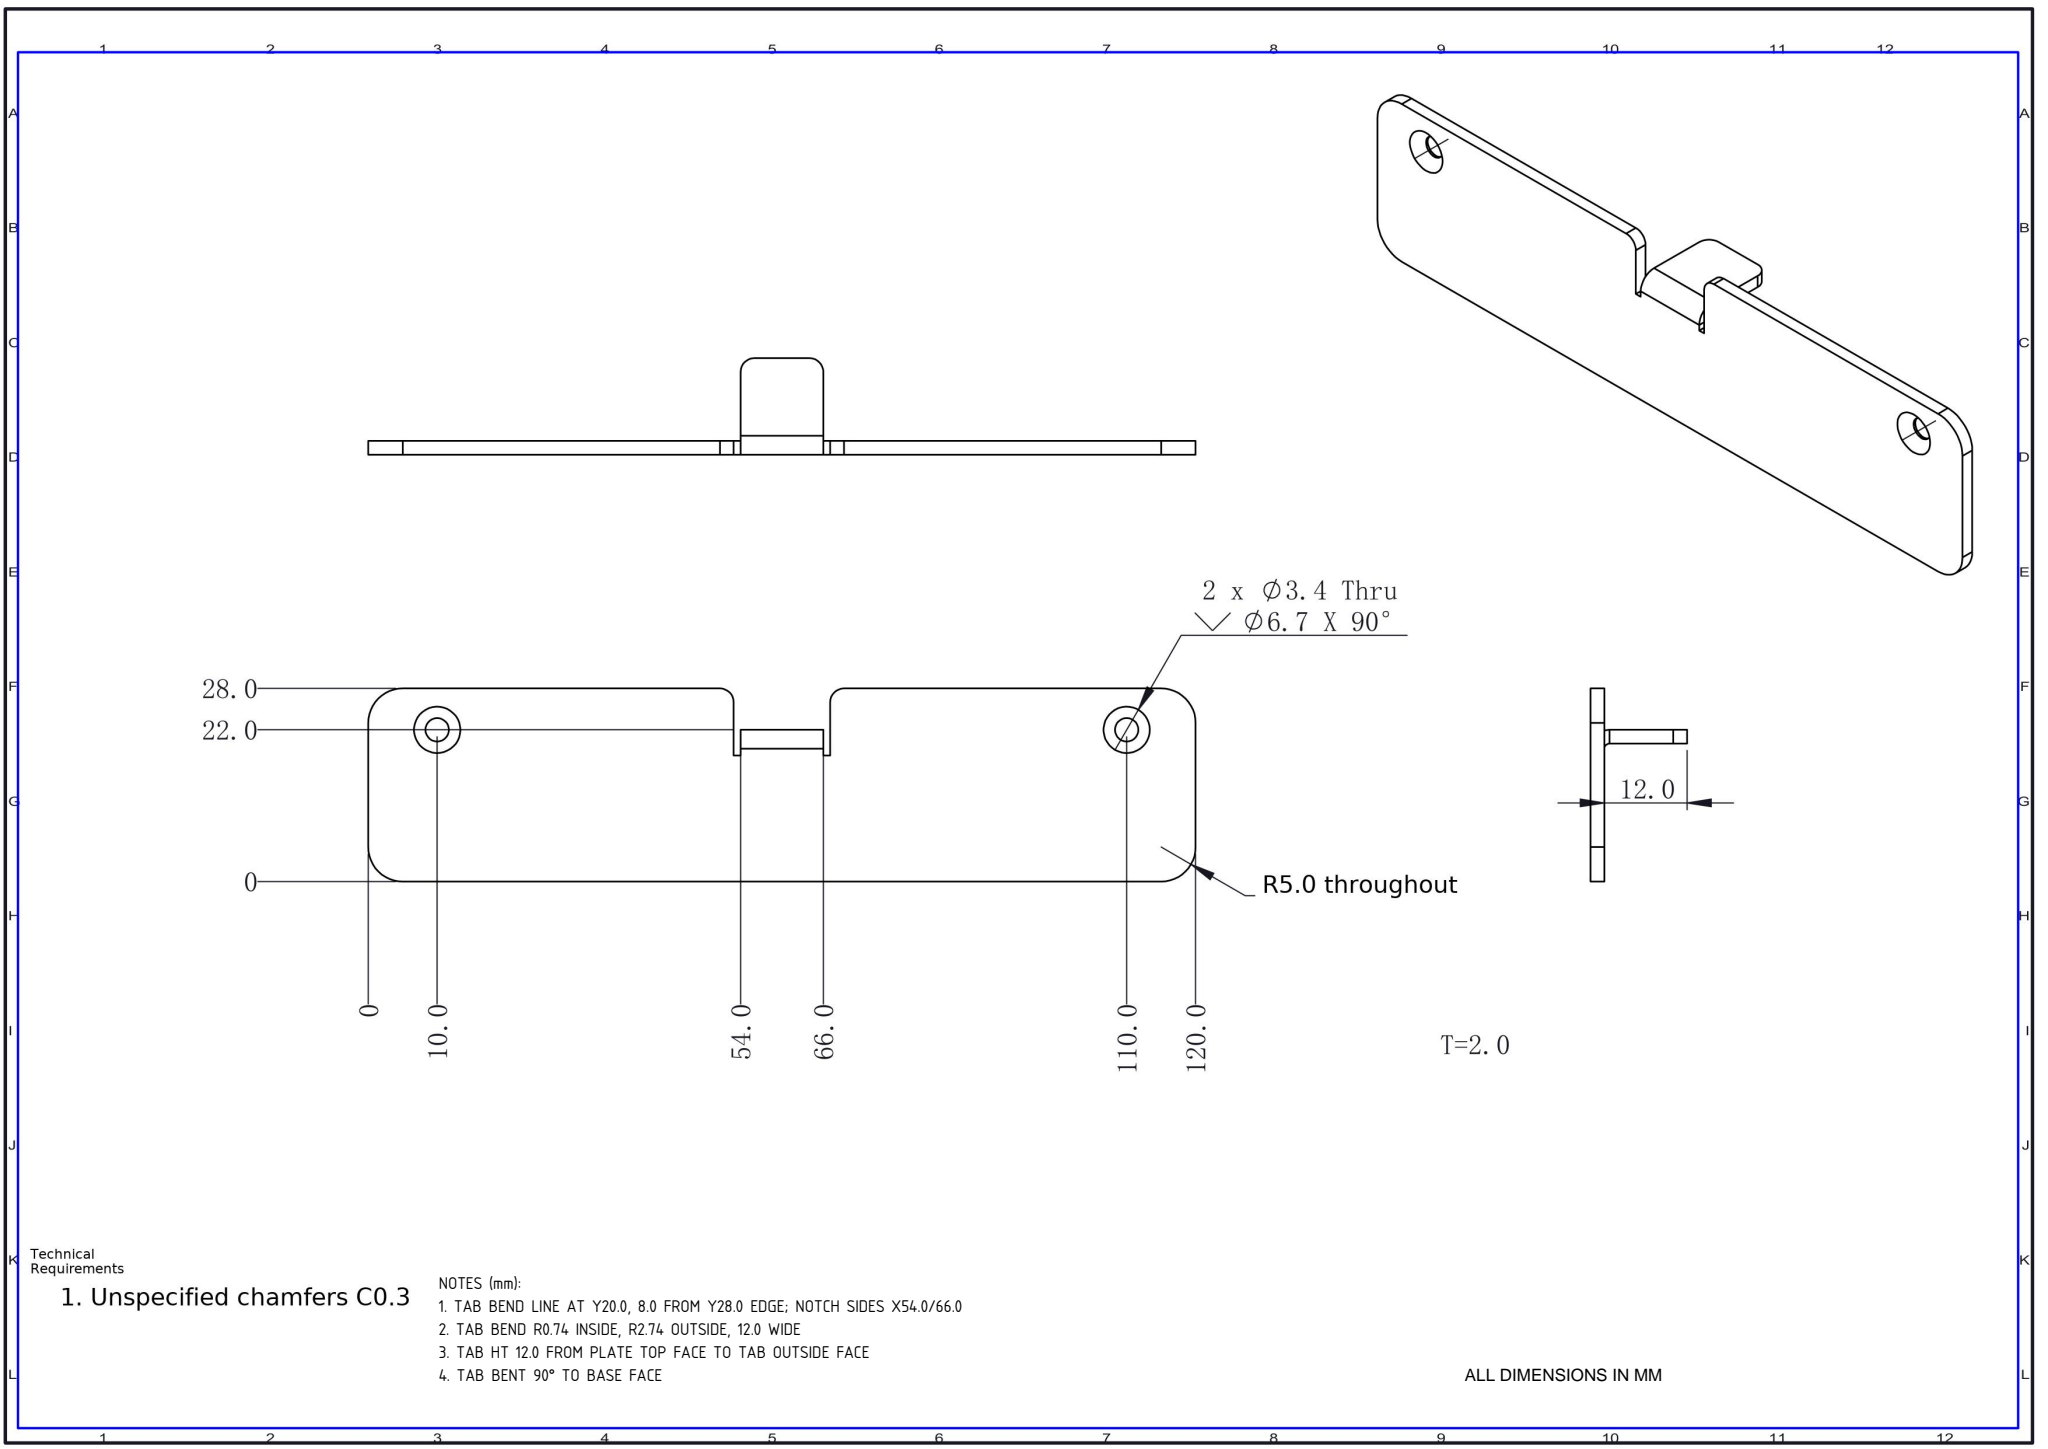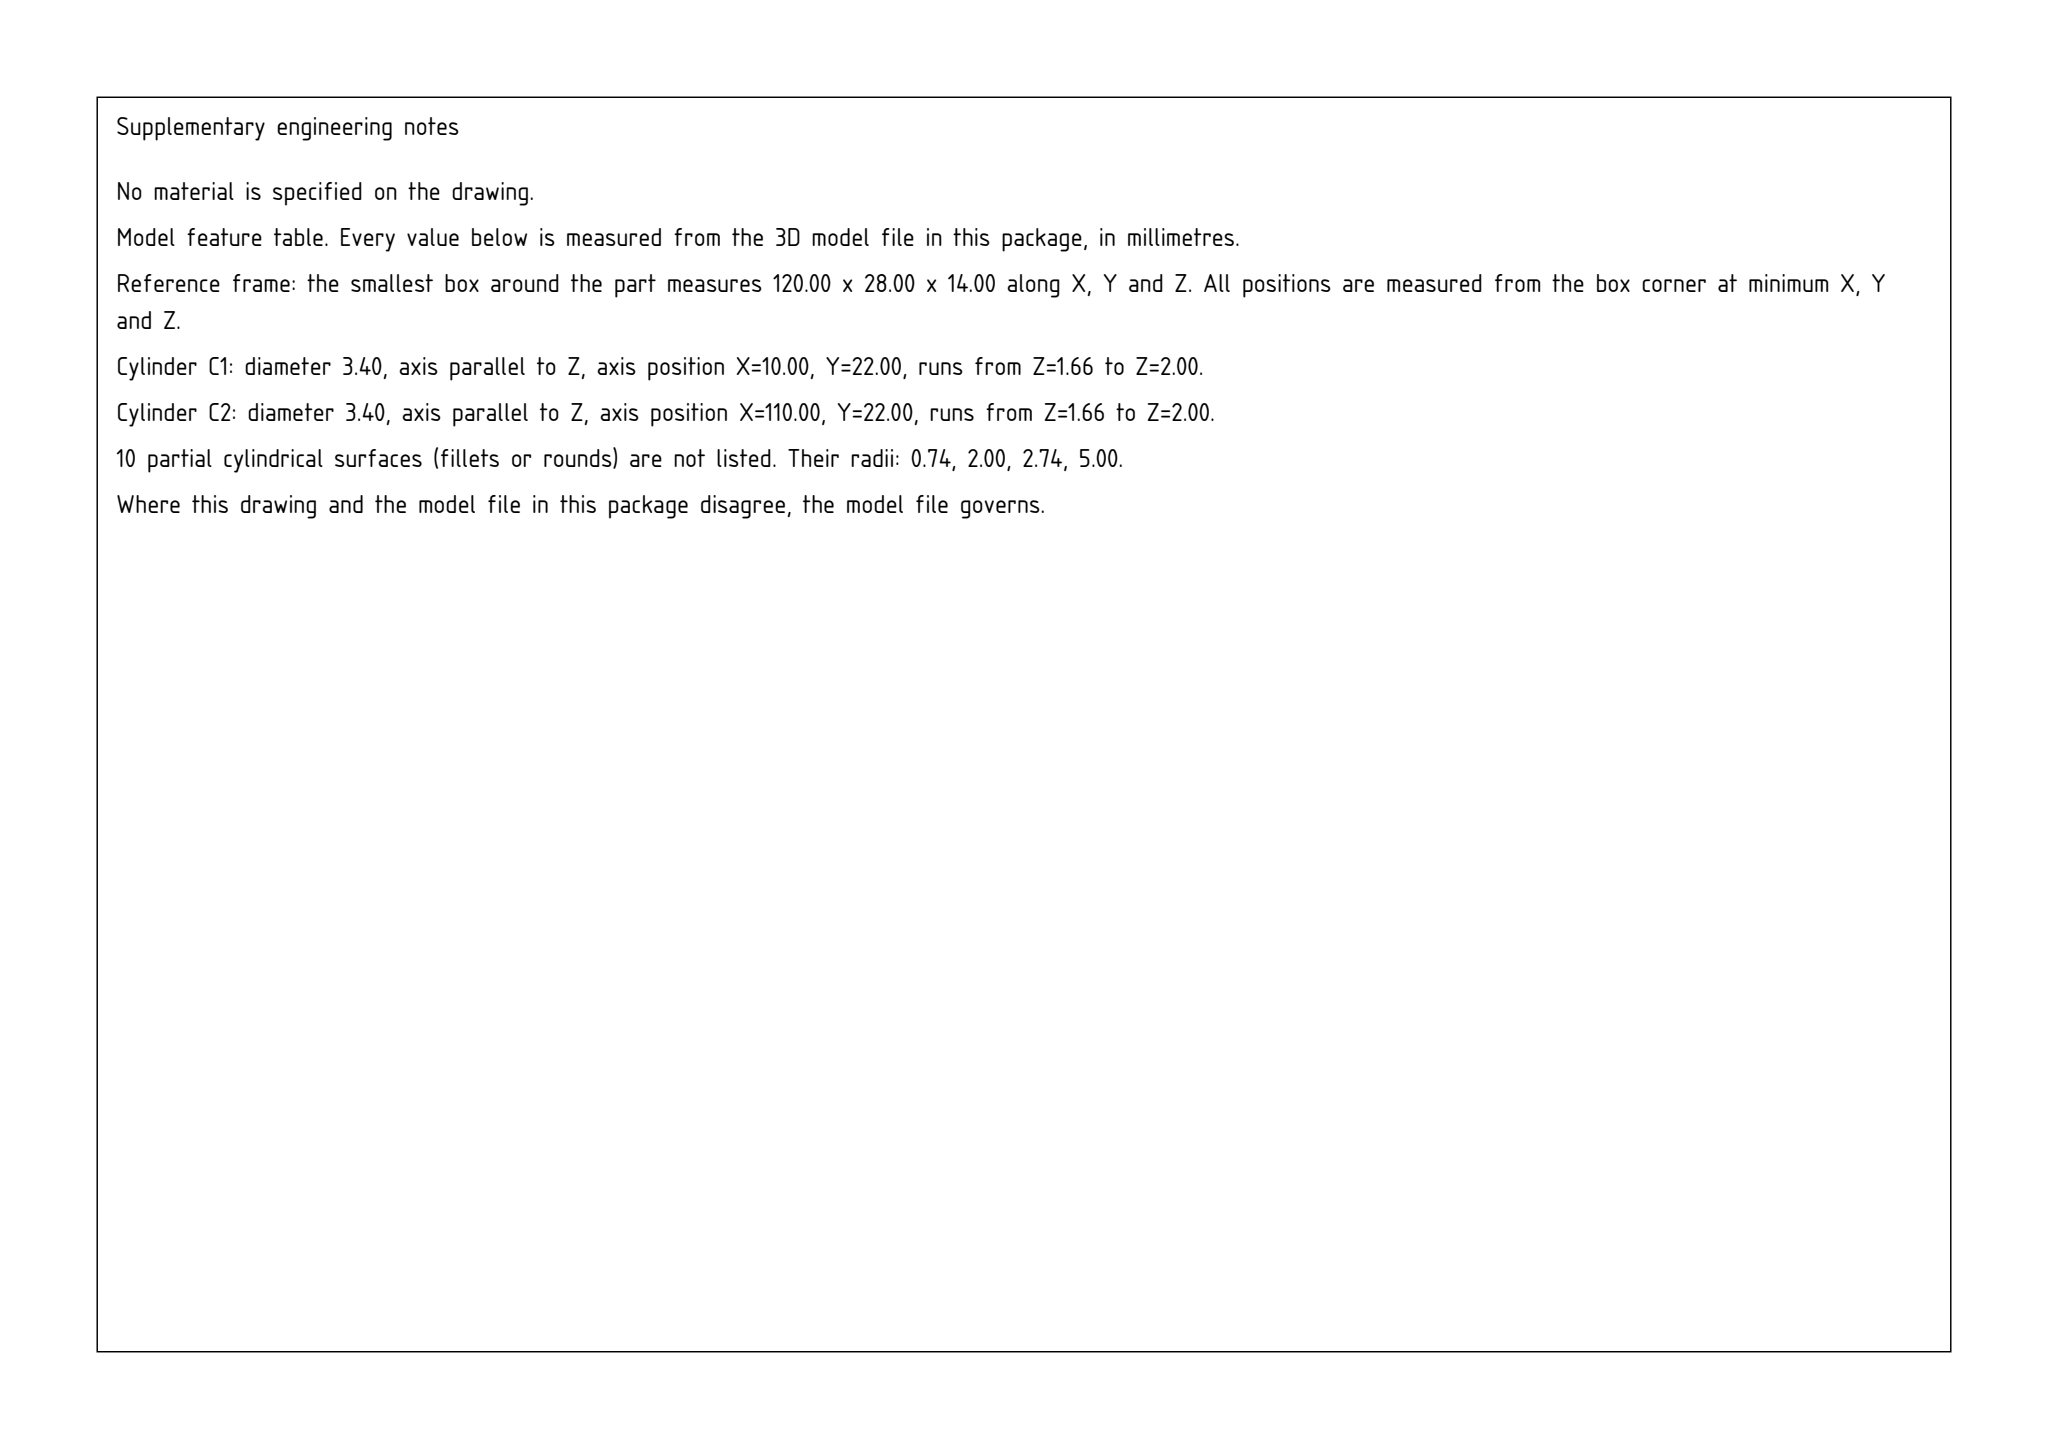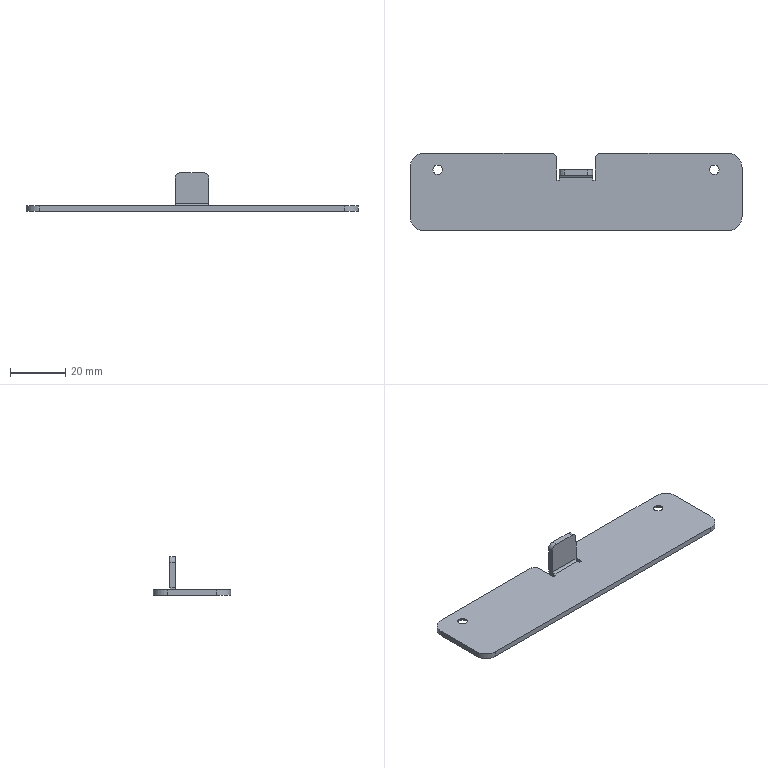Part | SolidWorks | mm | 1 solid | 38 faces | box 120 x 28 x 14 mm | volume 6682 mm3 | plane 20 | cylinder 14 | cone 4 | commonest cylinder face diameters 3.4 x4 10 x4 4 x4 5.473 x1 1.473 x1
Drawing notes:
TAB BEND LINE AT Y20.0, 8.0 FROM Y28.0 EDGE; NOTCH SIDES X54.0/66.0 | from the solid: axis_plane y=20.0 notch bottom edge; top edge y=28.0; planes x=54.0 and x=66.0
TAB BEND R0.74 INSIDE, R2.74 OUTSIDE, 12.0 WIDE | from the solid: cyls Ø1.473 & Ø5.473 about x-axis at y=19.26, z=2.74, len 12.0; 2.736-0.7365=2.0=T
TAB HT 12.0 FROM PLATE TOP FACE TO TAB OUTSIDE FACE | from the solid: plate faces z=0 and z=2.0; tab outer face z=14.0; 14.0-2.0=12.0
TAB BENT 90° TO BASE FACE | from the solid: Side and isometric views show upstand normal to 2.0 base plate; no STEP data supplied to confirm other angle